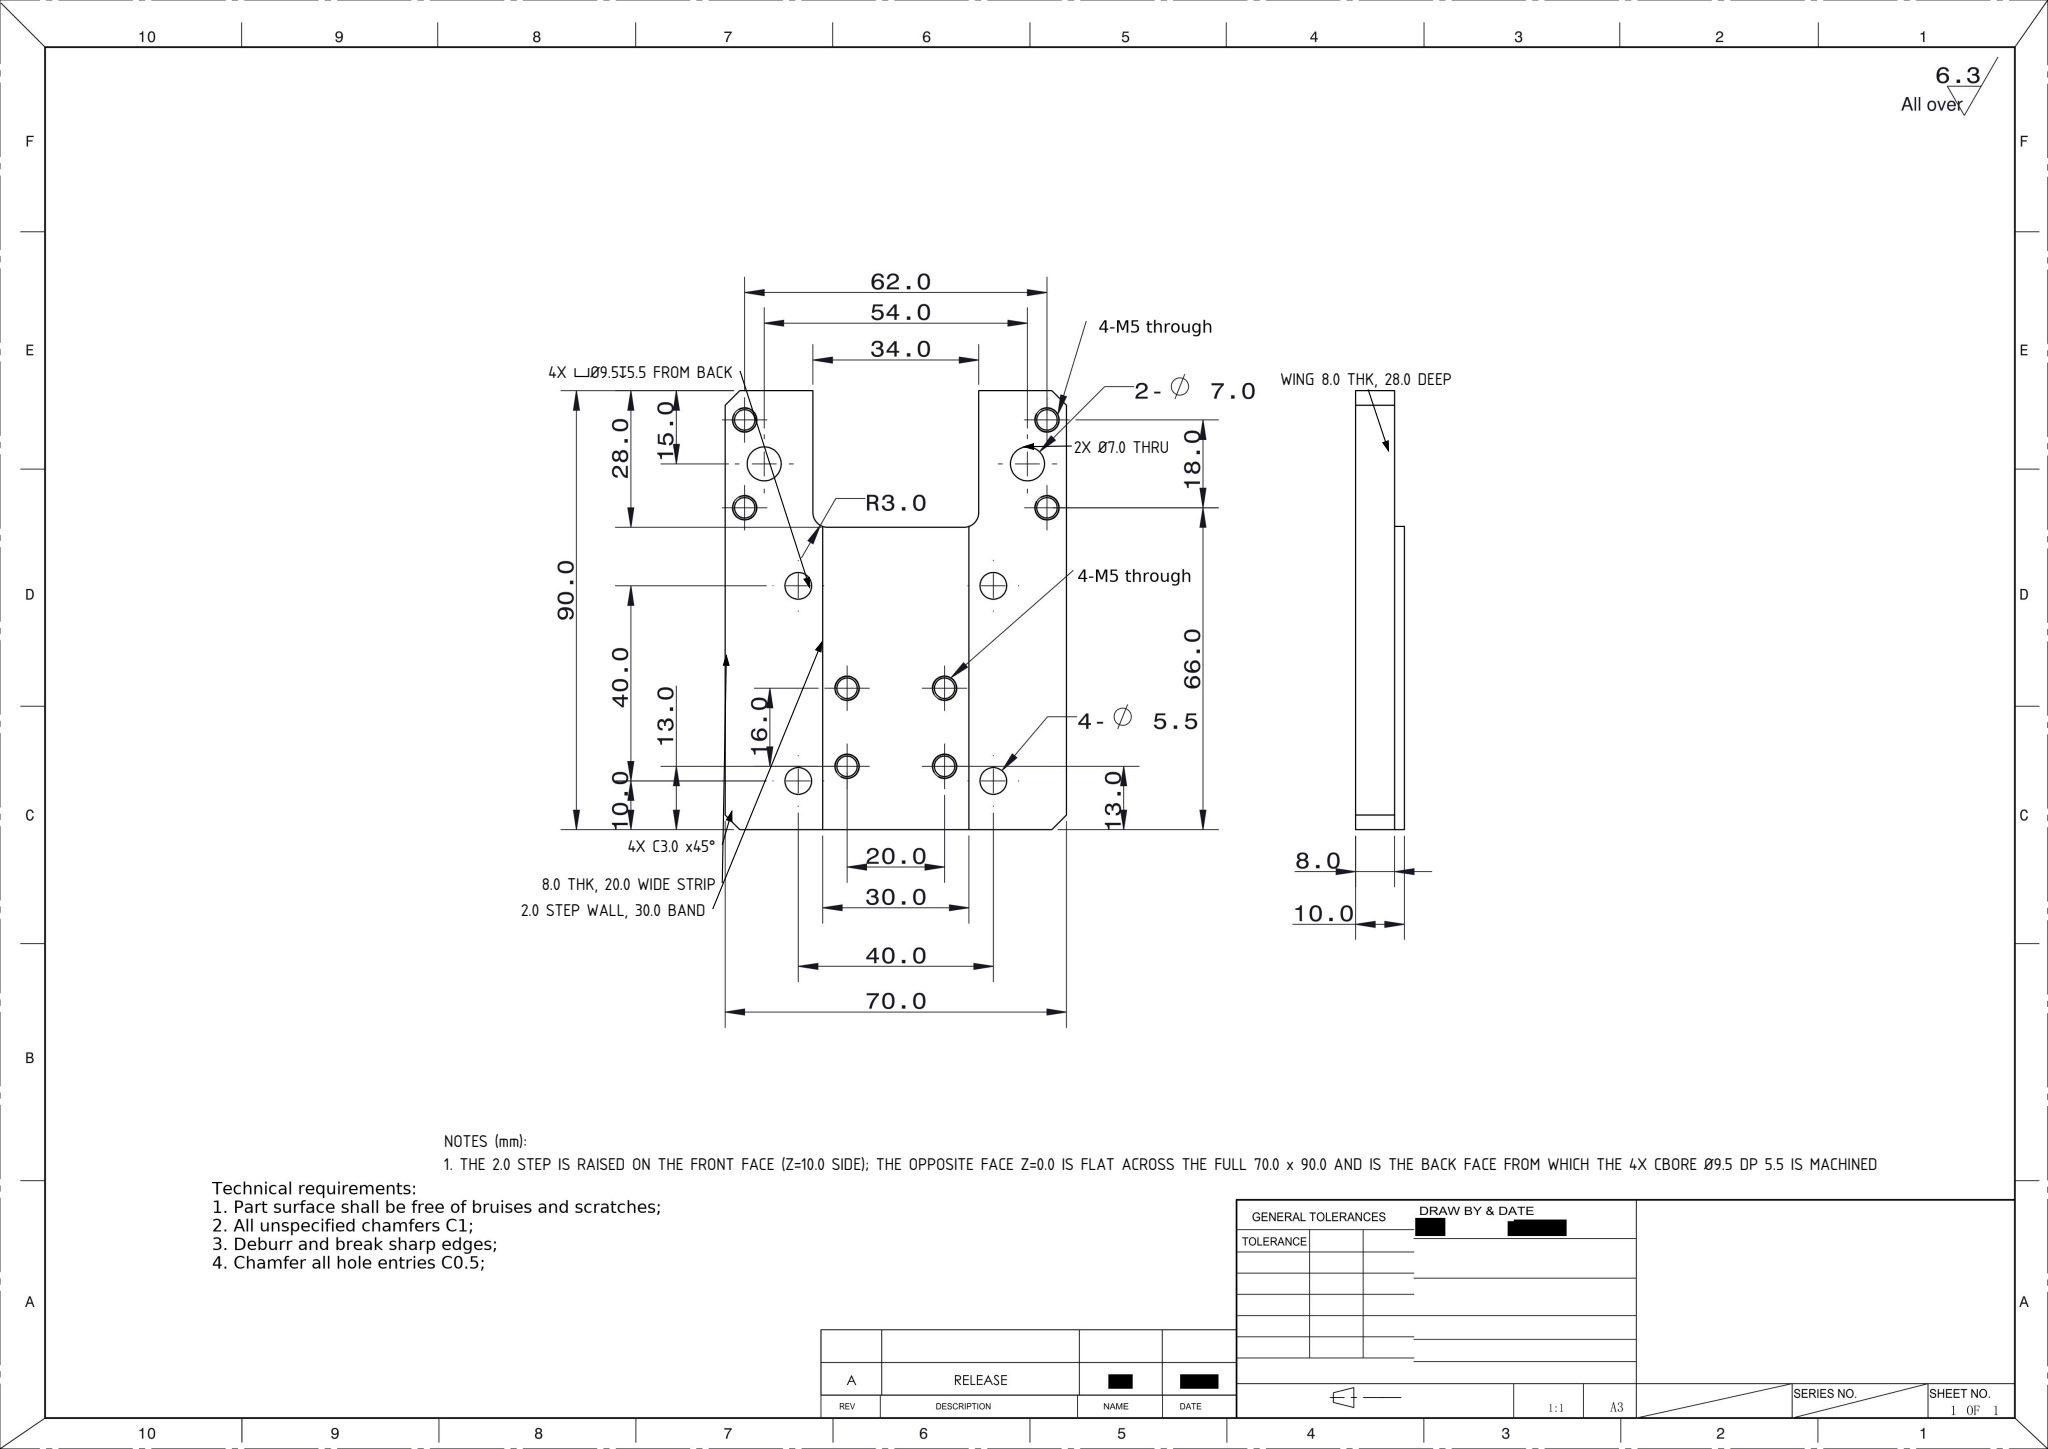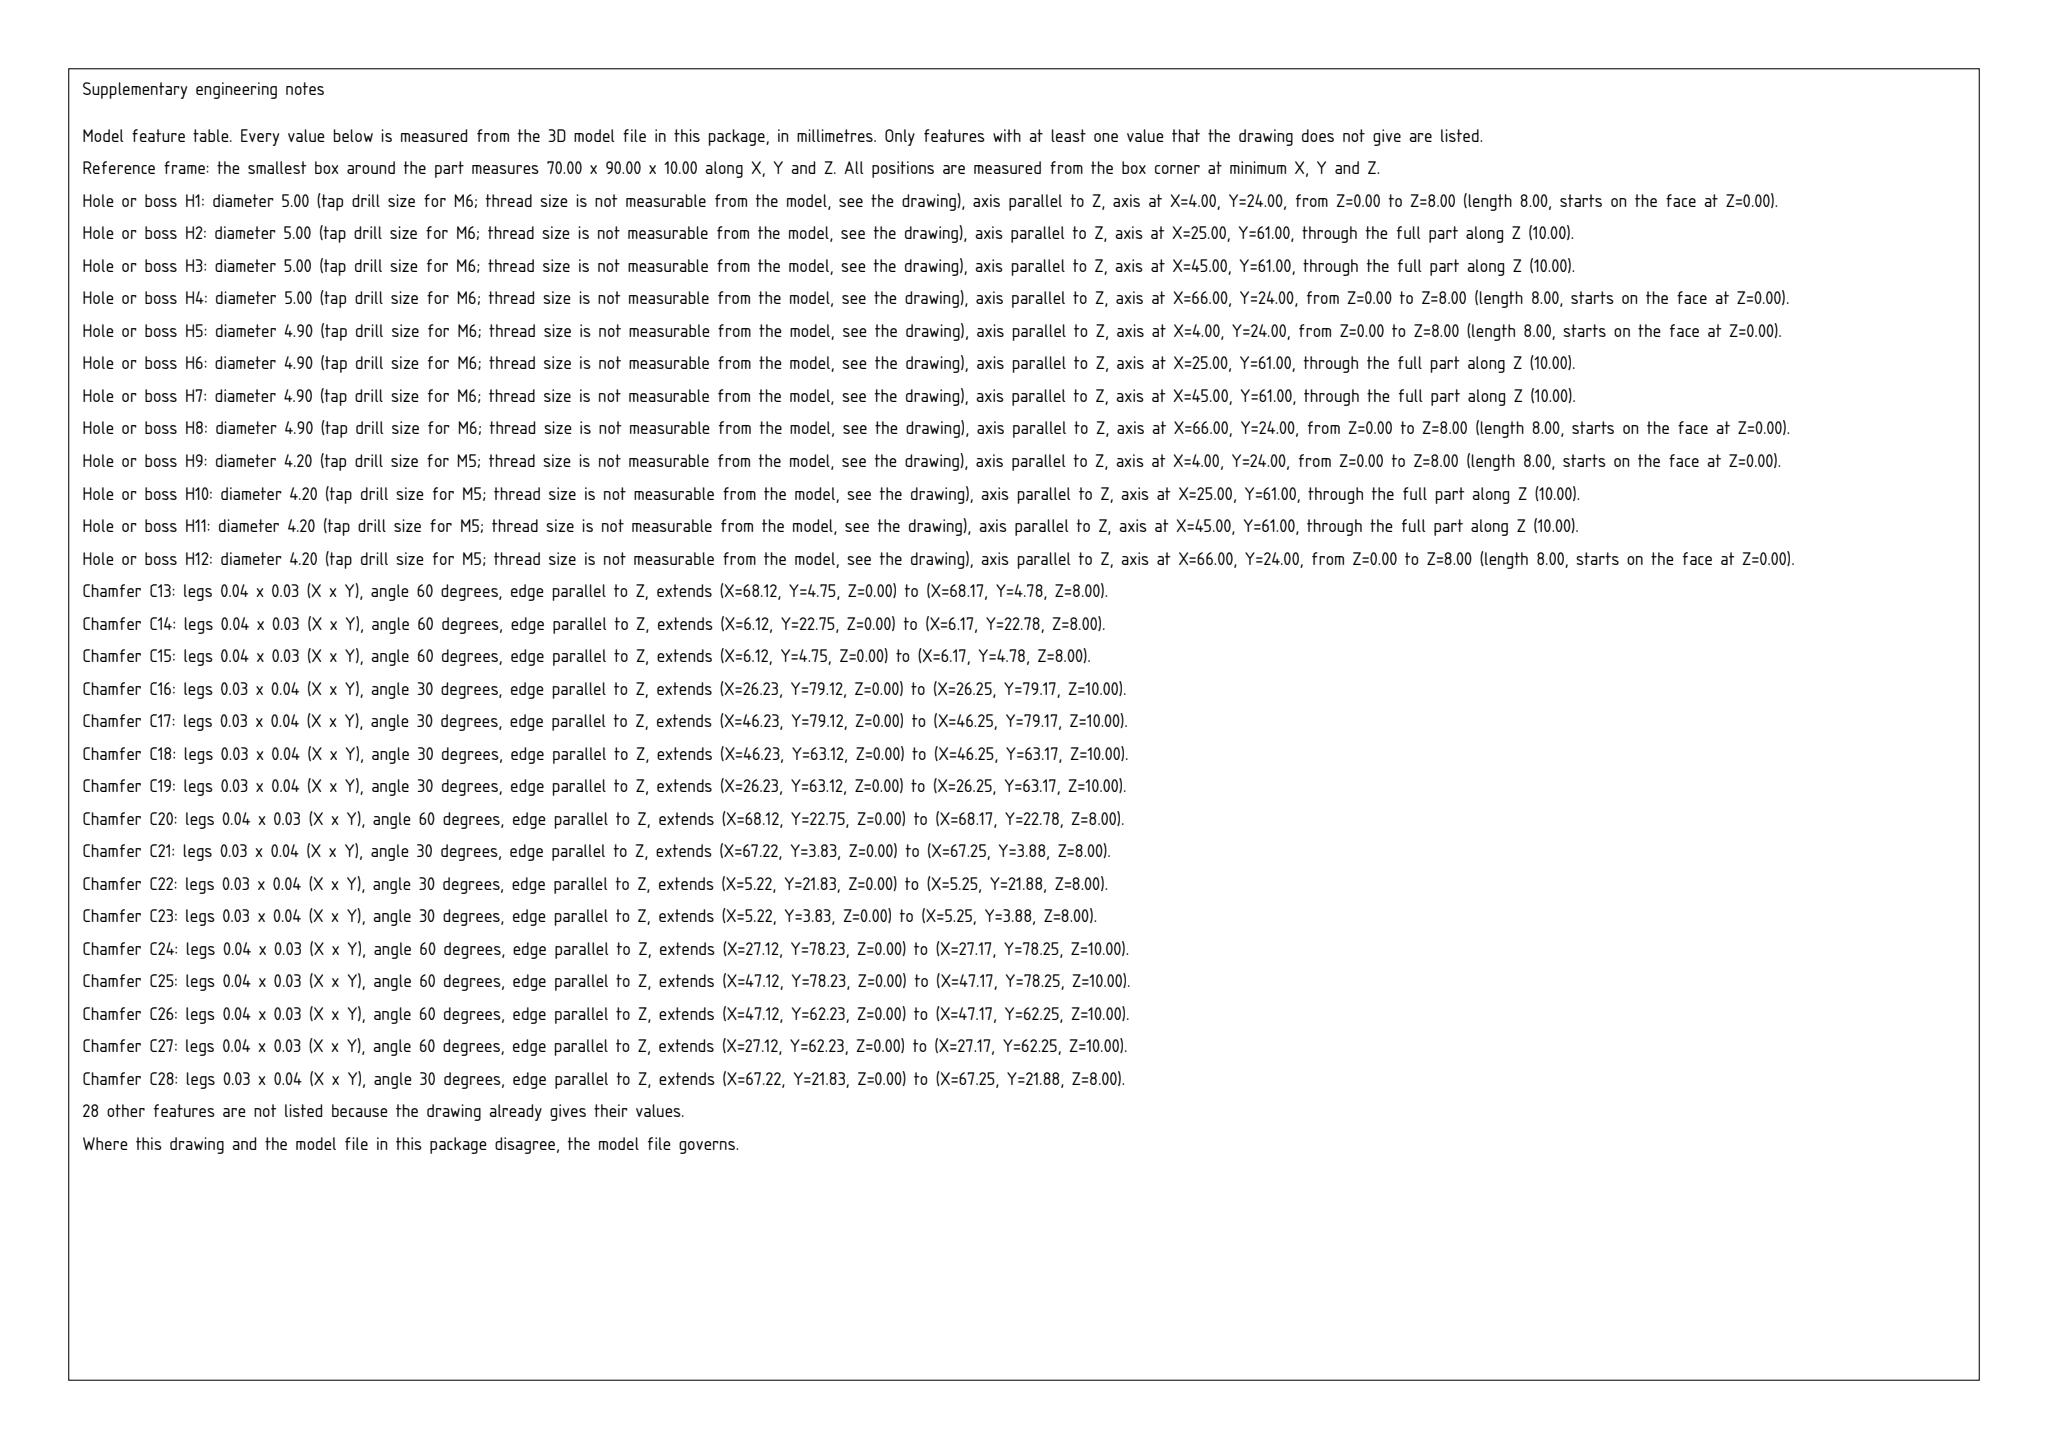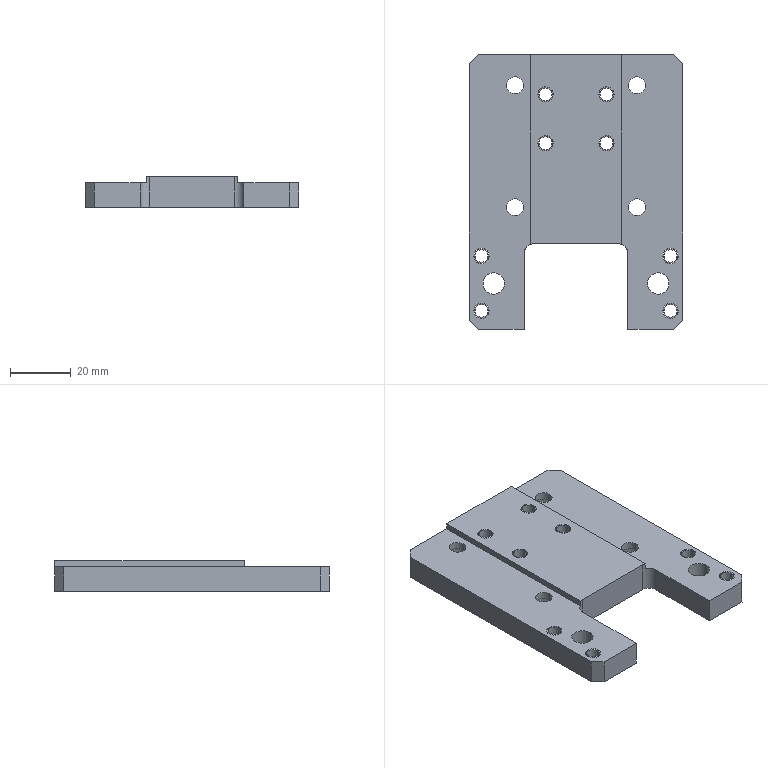Part | SolidWorks | mm | 1 solid | 124 faces | box 70 x 90 x 10 mm | volume 42930 mm3 | cylinder 86 | plane 38 | commonest cylinder face diameters 5 x24 4.9 x24 4.2 x16 9.5 x8 5.5 x8 7 x4 6 x2
Drawing notes:
TOP WINGS THK 8.0 (2.0 STEP), BOTH SIDES OF NOTCH, FULL 28.0 DEPTH | from the solid: z planes at 8.0 (x2); holes y=6/24 len 8.0 vs y=61/77 len 10.0; y plane 28.0; x planes 0-18 & 52-70
4-Ø5.5 THRU, CBORE Ø9.5 DP 5.5 FROM BACK FACE | from the solid: Ø9.5 z-cyls L=5.5 at (15,40),(15,80),(55,40),(55,80) coaxial with Ø5.5 L=2.5; z plane 5.5 x4
2-Ø7.0 THRU (8 THK WING) | from the solid: Ø7.0 z-cyls at (8,15) & (62,15), length 8.0 = wing thk (z planes 0 to 8.0)
4X CORNER CHAMFER 3.0 x 45° ON PLATE OUTLINE (AT CORNERS X0/Y0, X0/Y90, X70/Y0, X70/Y90 FROM LOWER-LEFT DATUM), FULL 8.0 THK WING HEIGHT - OVERRIDES GENERAL NOTE 'UNSPECIFIED CHAMFERS C1' | from the solid: inclined_planes angle_to_xyz_axes [45,45,90], bbox_from [0,0,0] / [0,87,0] / [67,0,0] / [67,87,0], size [3.0,3.0,8.0]
STEPPED THICKNESS: 20.0 WIDE SIDE STRIPS (X0.0-X20.0 AND X50.0-X70.0 FROM LOWER-LEFT DATUM) ARE 8.0 THK OVER THE FULL 90.0 LENGTH (Y0.0-Y90.0) | from the solid: axis_planes z=8.0 extent x[0,20] y[0,90] and x[50,70] y[0,90]
RAISED CENTRAL BAND 30.0 WIDE (X20.0 TO X50.0) IS 10.0 THK AND RUNS FROM THE NOTCH FACE Y28.0 TO THE Y90.0 EDGE (62.0 LONG); STEP WALLS AT X20.0 AND X50.0 ARE 2.0 HIGH | from the solid: axis_plane z=10.0 extent x[20,50] y[27.8,90]; axis_planes x=20.0 and x=50.0 extent y[27.8,90] z[8,10]
THE 2.0 STEP IS RAISED ON THE FRONT FACE (Z=10.0 SIDE); THE OPPOSITE FACE Z=0.0 IS FLAT ACROSS THE FULL 70.0 x 90.0 AND IS THE BACK FACE FROM WHICH THE 4X CBORE Ø9.5 DP 5.5 IS MACHINED | from the solid: axis_plane z=0.0 extent x[0,70] y[0,90]; hole/bore dia 9.5 from z 0.0 to 5.5 with dia 5.5 continuing z 5.5 to 8.0